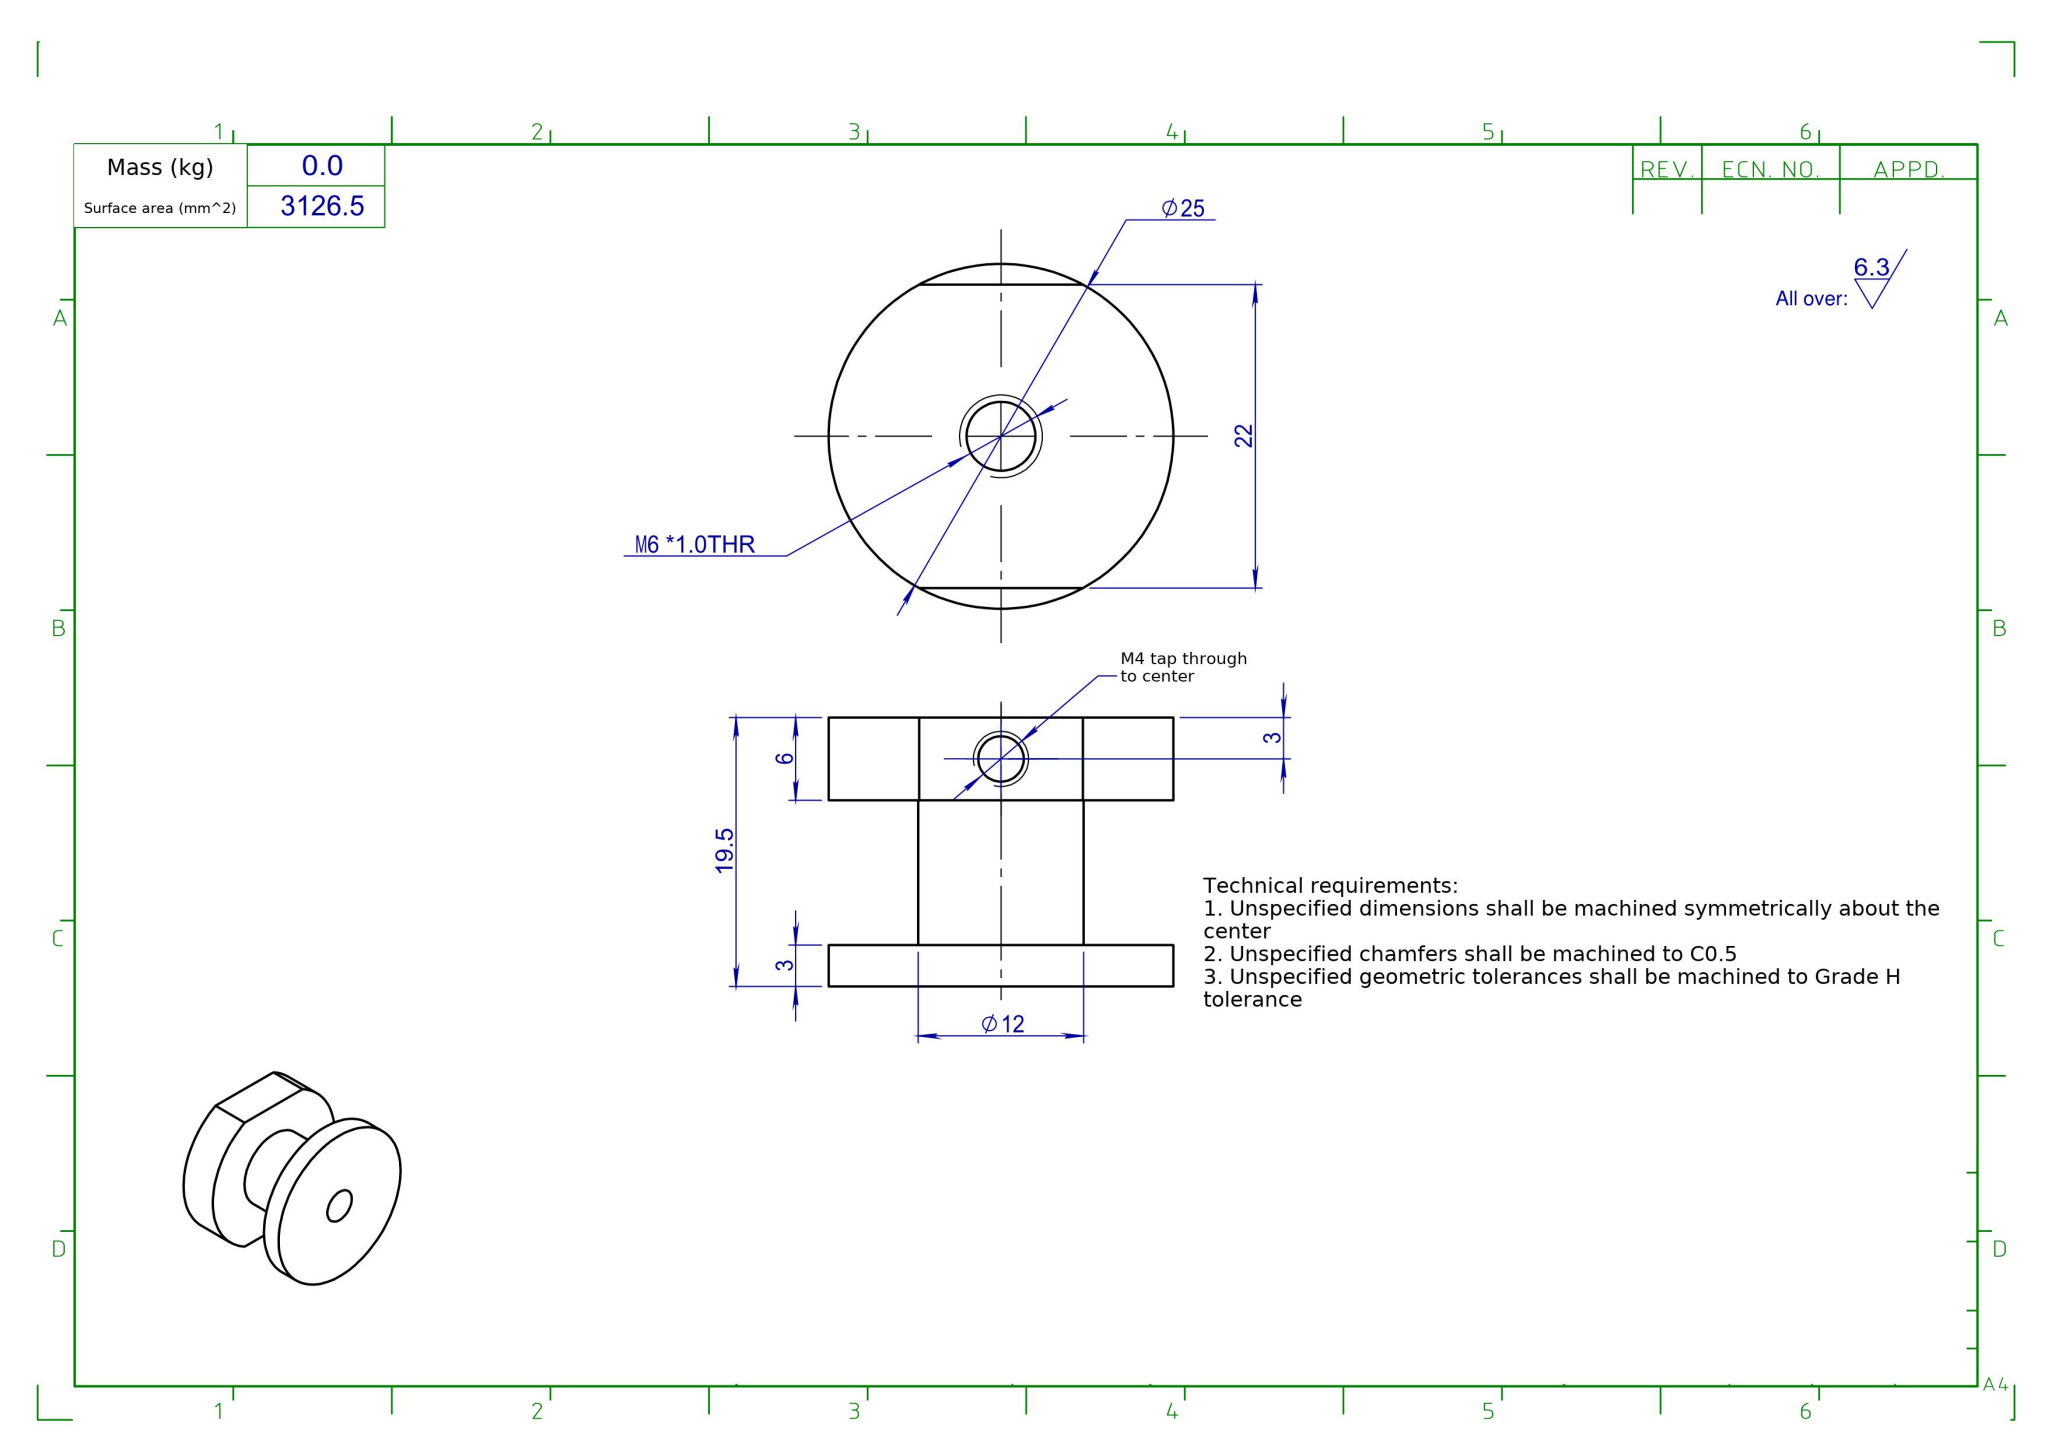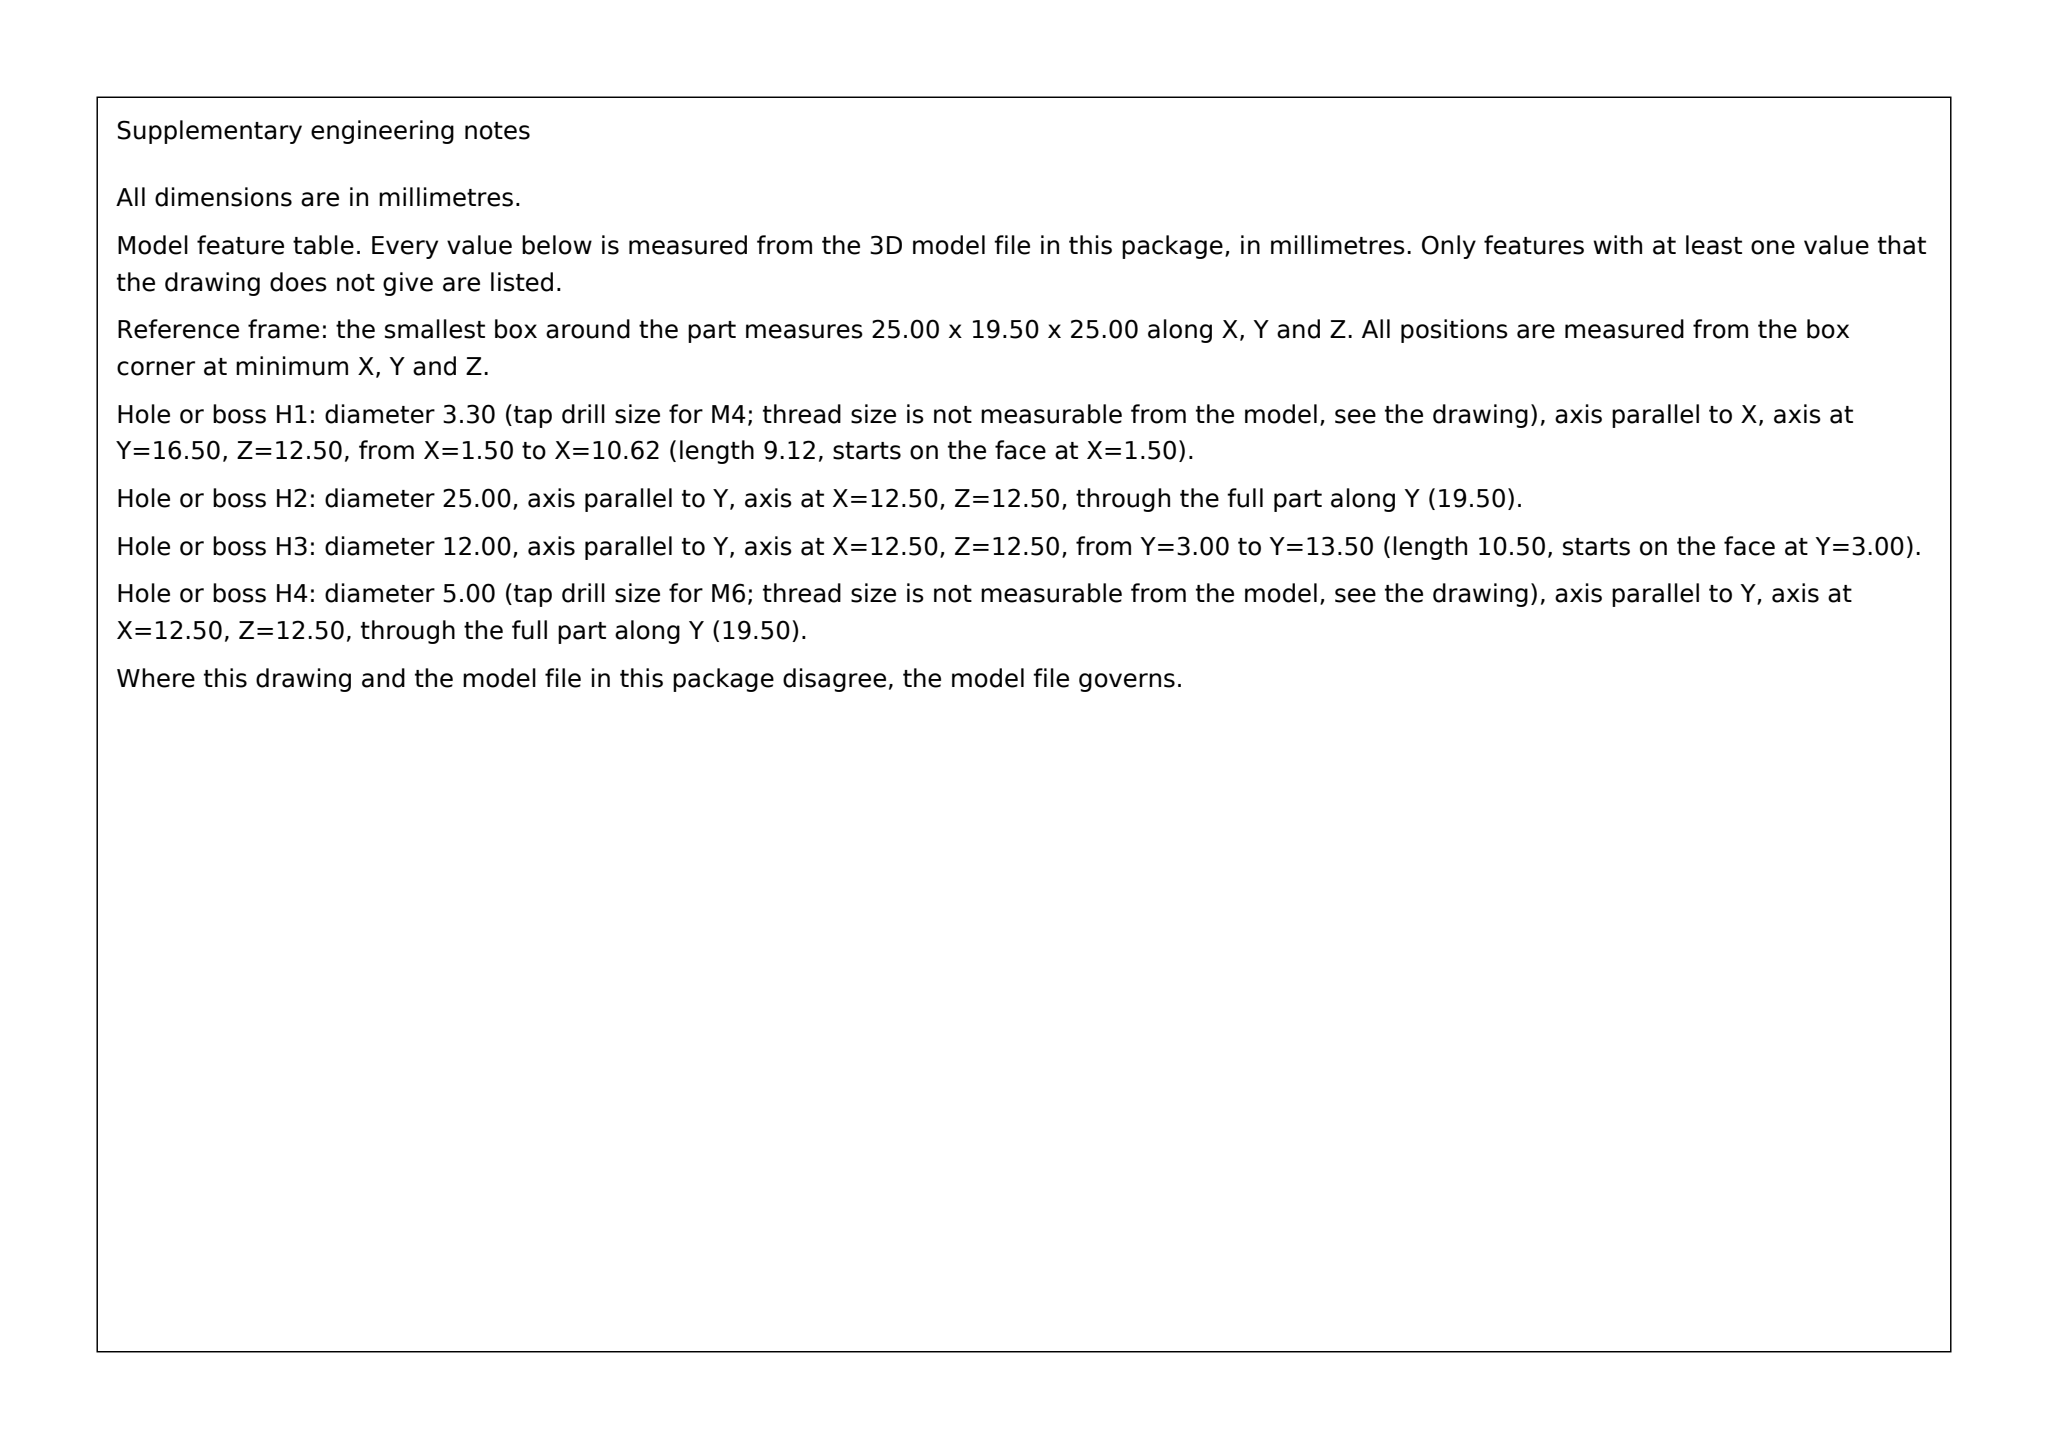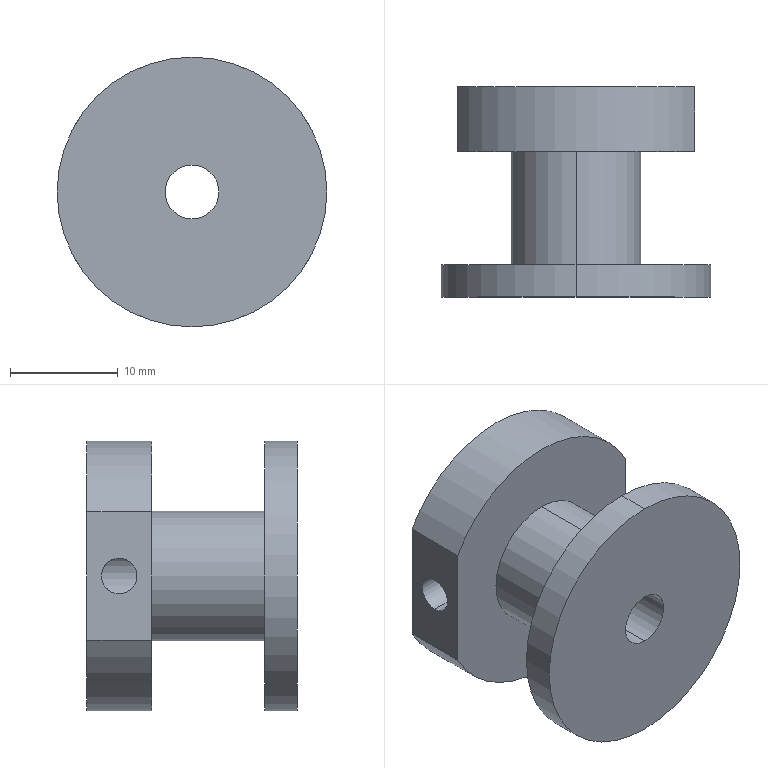Part | SolidWorks | mm | 1 solid | 17 faces | box 25 x 19.5 x 25 mm | volume 5004 mm3 | cylinder 11 | plane 6 | commonest cylinder face diameters 25 x5 3.3 x2 5 x2 12 x2
STEP:
#1=CARTESIAN_POINT('',(-1.878,16.5,-1.65));
#2=VERTEX_POINT('',#1);
#3=CARTESIAN_POINT('',(-1.878,16.5,1.65));
#4=VERTEX_POINT('',#3);
#5=CARTESIAN_POINT('',(-1.878,16.5,-1.65));
#6=CARTESIAN_POINT('',(-1.878,16.277,-1.65));
#7=CARTESIAN_POINT('',(-1.921,16.056,-1.603));
#8=CARTESIAN_POINT('',(-2.049,15.661,-1.437));
#9=CARTESIAN_POINT('',(-2.131,15.485,-1.318));
#10=CARTESIAN_POINT('',(-2.249,15.262,-1.096));
#11=CARTESIAN_POINT('',(-2.286,15.195,-1.016));
#12=CARTESIAN_POINT('',(-2.356,15.077,-0.8415));
#13=CARTESIAN_POINT('',(-2.388,15.025,-0.7465));
#14=CARTESIAN_POINT('',(-2.442,14.939,-0.5467));
#15=CARTESIAN_POINT('',(-2.463,14.907,-0.4426));
#16=CARTESIAN_POINT('',(-2.492,14.862,-0.2252));
#17=CARTESIAN_POINT('',(-2.5,14.85,-0.113));
#18=CARTESIAN_POINT('',(-2.5,14.85,0.109));
#19=CARTESIAN_POINT('',(-2.493,14.861,0.2216));
#20=CARTESIAN_POINT('',(-2.464,14.906,0.439));
#21=CARTESIAN_POINT('',(-2.442,14.938,0.5434));
#22=CARTESIAN_POINT('',(-2.362,15.066,0.8448));
#23=CARTESIAN_POINT('',(-2.288,15.188,1.022));
#24=CARTESIAN_POINT('',(-2.17,15.41,1.243));
#25=CARTESIAN_POINT('',(-2.131,15.491,1.31));
#26=CARTESIAN_POINT('',(-2.054,15.665,1.427));
#27=CARTESIAN_POINT('',(-2.017,15.759,1.478));
#28=CARTESIAN_POINT('',(-1.922,16.053,1.603));
#29=CARTESIAN_POINT('',(-1.878,16.275,1.65));
#30=CARTESIAN_POINT('',(-1.878,16.5,1.65));
#31=B_SPLINE_CURVE_WITH_KNOTS('',3,(#5,#6,#7,#8,#9,#10,#11,#12,#13,#14,#15,#16,#17,#18,#19,#20,#21,#22,#23,#24,#25,#26,#27,#28,#29,#30),.UNSPECIFIED.,.F.,.F.,(4,2,2,2,2,2,2,2,2,2,2,2,4),(0.005325,0.005989,0.006652,0.006984,0.007316,0.007648,0.00798,0.008311,0.008643,0.009307,0.009639,0.00997,0.01063),.UNSPECIFIED.);
#32=EDGE_CURVE('',#2,#4,#31,.T.);
#33=ORIENTED_EDGE('',*,*,#32,.F.);
#34=CARTESIAN_POINT('',(-11.,16.5,-1.65));
#35=VERTEX_POINT('',#34);
#36=CARTESIAN_POINT('',(-11.,16.5,-1.65));
#37=DIRECTION('',(-1.,0.,-0.));
#38=VECTOR('',#37,1000.);
#39=LINE('',#36,#38);
#40=EDGE_CURVE('',#2,#35,#39,.T.);
#41=ORIENTED_EDGE('',*,*,#40,.T.);
#42=CARTESIAN_POINT('',(-11.,16.5,1.65));
#43=VERTEX_POINT('',#42);
#44=CARTESIAN_POINT('',(-11.,16.5,-0.));
#45=DIRECTION('',(-1.,0.,-0.));
#46=DIRECTION('',(0.,0.,1.));
#47=AXIS2_PLACEMENT_3D('',#44,#45,#46);
#48=CIRCLE('',#47,1.65);
#49=EDGE_CURVE('',#35,#43,#48,.T.);
#50=ORIENTED_EDGE('',*,*,#49,.T.);
#51=CARTESIAN_POINT('',(-11.,16.5,1.65));
#52=DIRECTION('',(-1.,0.,-0.));
#53=VECTOR('',#52,1000.);
#54=LINE('',#51,#53);
#55=EDGE_CURVE('',#4,#43,#54,.T.);
#56=ORIENTED_EDGE('',*,*,#55,.F.);
#57=EDGE_LOOP('',(#33,#41,#50,#56));
#58=FACE_OUTER_BOUND('',#57,.T.);
#59=CARTESIAN_POINT('',(-11.,16.5,-0.));
#60=DIRECTION('',(-1.,0.,-0.));
#61=DIRECTION('',(0.,0.,1.));
#62=AXIS2_PLACEMENT_3D('',#59,#60,#61);
#63=CYLINDRICAL_SURFACE('',#62,1.65);
#64=ADVANCED_FACE('',(#58),#63,.F.);
#65=CARTESIAN_POINT('',(-1.878,16.5,1.65));
#66=CARTESIAN_POINT('',(-1.878,16.613,1.65));
#67=CARTESIAN_POINT('',(-1.888,16.723,1.639));
#68=CARTESIAN_POINT('',(-1.926,16.938,1.595));
#69=CARTESIAN_POINT('',(-1.953,17.043,1.562));
#70=CARTESIAN_POINT('',(-2.048,17.339,1.437));
#71=CARTESIAN_POINT('',(-2.131,17.515,1.318));
#72=CARTESIAN_POINT('',(-2.248,17.737,1.097));
#73=CARTESIAN_POINT('',(-2.287,17.805,1.015));
#74=CARTESIAN_POINT('',(-2.356,17.924,0.8403));
#75=CARTESIAN_POINT('',(-2.388,17.975,0.7473));
#76=CARTESIAN_POINT('',(-2.441,18.06,0.5487));
#77=CARTESIAN_POINT('',(-2.463,18.094,0.4419));
#78=CARTESIAN_POINT('',(-2.492,18.138,0.2266));
#79=CARTESIAN_POINT('',(-2.5,18.15,0.1166));
#80=CARTESIAN_POINT('',(-2.5,18.151,-0.2205));
#81=CARTESIAN_POINT('',(-2.469,18.104,-0.4434));
#82=CARTESIAN_POINT('',(-2.363,17.935,-0.8431));
#83=CARTESIAN_POINT('',(-2.288,17.813,-1.021));
#84=CARTESIAN_POINT('',(-2.171,17.59,-1.243));
#85=CARTESIAN_POINT('',(-2.13,17.508,-1.31));
#86=CARTESIAN_POINT('',(-2.054,17.335,-1.427));
#87=CARTESIAN_POINT('',(-2.017,17.243,-1.477));
#88=CARTESIAN_POINT('',(-1.922,16.947,-1.603));
#89=CARTESIAN_POINT('',(-1.878,16.724,-1.65));
#90=CARTESIAN_POINT('',(-1.878,16.5,-1.65));
#91=B_SPLINE_CURVE_WITH_KNOTS('',3,(#65,#66,#67,#68,#69,#70,#71,#72,#73,#74,#75,#76,#77,#78,#79,#80,#81,#82,#83,#84,#85,#86,#87,#88,#89,#90),.UNSPECIFIED.,.F.,.F.,(4,2,2,2,2,2,2,2,2,2,2,2,4),(0.,0.0003328,0.0006656,0.001331,0.001664,0.001997,0.00233,0.002663,0.003328,0.003994,0.004327,0.004659,0.005325),.UNSPECIFIED.);
#92=EDGE_CURVE('',#4,#2,#91,.T.);
#93=ORIENTED_EDGE('',*,*,#92,.T.);
#94=ORIENTED_EDGE('',*,*,#32,.T.);
#95=EDGE_LOOP('',(#93,#94));
#96=FACE_BOUND('',#95,.T.);
#97=CARTESIAN_POINT('',(0.,0.,-2.5));
#98=VERTEX_POINT('',#97);
#99=CARTESIAN_POINT('',(0.,0.,2.5));
#100=VERTEX_POINT('',#99);
#101=CARTESIAN_POINT('',(0.,0.,0.));
#102=DIRECTION('',(0.,1.,0.));
#103=DIRECTION('',(0.,0.,1.));
#104=AXIS2_PLACEMENT_3D('',#101,#102,#103);
#105=CIRCLE('',#104,2.5);
#106=EDGE_CURVE('',#98,#100,#105,.T.);
#107=ORIENTED_EDGE('',*,*,#106,.F.);
#108=CARTESIAN_POINT('',(0.,19.5,-2.5));
#109=VERTEX_POINT('',#108);
#110=CARTESIAN_POINT('',(0.,19.5,-2.5));
#111=DIRECTION('',(0.,1.,0.));
#112=VECTOR('',#111,1000.);
#113=LINE('',#110,#112);
#114=EDGE_CURVE('',#98,#109,#113,.T.);
#115=ORIENTED_EDGE('',*,*,#114,.T.);
#116=CARTESIAN_POINT('',(0.,19.5,2.5));
#117=VERTEX_POINT('',#116);
#118=CARTESIAN_POINT('',(0.,19.5,0.));
#119=DIRECTION('',(0.,1.,0.));
#120=DIRECTION('',(0.,0.,1.));
#121=AXIS2_PLACEMENT_3D('',#118,#119,#120);
#122=CIRCLE('',#121,2.5);
#123=EDGE_CURVE('',#109,#117,#122,.T.);
#124=ORIENTED_EDGE('',*,*,#123,.T.);
#125=CARTESIAN_POINT('',(0.,19.5,2.5));
#126=DIRECTION('',(0.,1.,0.));
#127=VECTOR('',#126,1000.);
#128=LINE('',#125,#127);
#129=EDGE_CURVE('',#100,#117,#128,.T.);
#130=ORIENTED_EDGE('',*,*,#129,.F.);
#131=EDGE_LOOP('',(#107,#115,#124,#130));
#132=FACE_OUTER_BOUND('',#131,.T.);
#133=CARTESIAN_POINT('',(0.,19.5,0.));
#134=DIRECTION('',(0.,1.,0.));
#135=DIRECTION('',(0.,0.,1.));
#136=AXIS2_PLACEMENT_3D('',#133,#134,#135);
#137=CYLINDRICAL_SURFACE('',#136,2.5);
#138=ADVANCED_FACE('',(#96,#132),#137,.F.);
#139=CARTESIAN_POINT('',(0.,13.5,6.));
#140=VERTEX_POINT('',#139);
#141=CARTESIAN_POINT('',(0.,13.5,-6.));
#142=VERTEX_POINT('',#141);
#143=CARTESIAN_POINT('',(0.,13.5,0.));
#144=DIRECTION('',(0.,1.,0.));
#145=DIRECTION('',(0.,0.,1.));
#146=AXIS2_PLACEMENT_3D('',#143,#144,#145);
#147=CIRCLE('',#146,6.);
#148=EDGE_CURVE('',#140,#142,#147,.T.);
#149=ORIENTED_EDGE('',*,*,#148,.F.);
#150=CARTESIAN_POINT('',(0.,3.,6.));
#151=VERTEX_POINT('',#150);
#152=CARTESIAN_POINT('',(0.,13.5,6.));
#153=DIRECTION('',(0.,-1.,0.));
#154=VECTOR('',#153,1000.);
#155=LINE('',#152,#154);
#156=EDGE_CURVE('',#140,#151,#155,.T.);
#157=ORIENTED_EDGE('',*,*,#156,.T.);
#158=CARTESIAN_POINT('',(0.,3.,-6.));
#159=VERTEX_POINT('',#158);
#160=CARTESIAN_POINT('',(0.,3.,0.));
#161=DIRECTION('',(0.,1.,0.));
#162=DIRECTION('',(0.,0.,1.));
#163=AXIS2_PLACEMENT_3D('',#160,#161,#162);
#164=CIRCLE('',#163,6.);
#165=EDGE_CURVE('',#151,#159,#164,.T.);
#166=ORIENTED_EDGE('',*,*,#165,.T.);
#167=CARTESIAN_POINT('',(0.,13.5,-6.));
#168=DIRECTION('',(0.,-1.,0.));
#169=VECTOR('',#168,1000.);
#170=LINE('',#167,#169);
#171=EDGE_CURVE('',#142,#159,#170,.T.);
#172=ORIENTED_EDGE('',*,*,#171,.F.);
#173=EDGE_LOOP('',(#149,#157,#166,#172));
#174=FACE_OUTER_BOUND('',#173,.T.);
#175=CARTESIAN_POINT('',(0.,13.5,0.));
#176=DIRECTION('',(0.,-1.,0.));
#177=DIRECTION('',(0.,0.,-1.));
#178=AXIS2_PLACEMENT_3D('',#175,#176,#177);
#179=CYLINDRICAL_SURFACE('',#178,6.);
#180=ADVANCED_FACE('',(#174),#179,.T.);
#181=CARTESIAN_POINT('',(0.,3.,12.5));
#182=VERTEX_POINT('',#181);
#183=CARTESIAN_POINT('',(0.,3.,-12.5));
#184=VERTEX_POINT('',#183);
#185=CARTESIAN_POINT('',(0.,3.,0.));
#186=DIRECTION('',(0.,1.,0.));
#187=DIRECTION('',(0.,0.,1.));
#188=AXIS2_PLACEMENT_3D('',#185,#186,#187);
#189=CIRCLE('',#188,12.5);
#190=EDGE_CURVE('',#182,#184,#189,.T.);
#191=ORIENTED_EDGE('',*,*,#190,.F.);
#192=CARTESIAN_POINT('',(0.,0.,12.5));
#193=VERTEX_POINT('',#192);
#194=CARTESIAN_POINT('',(0.,3.,12.5));
#195=DIRECTION('',(0.,-1.,0.));
#196=VECTOR('',#195,1000.);
#197=LINE('',#194,#196);
#198=EDGE_CURVE('',#182,#193,#197,.T.);
#199=ORIENTED_EDGE('',*,*,#198,.T.);
#200=CARTESIAN_POINT('',(0.,0.,-12.5));
#201=VERTEX_POINT('',#200);
#202=CARTESIAN_POINT('',(0.,0.,0.));
#203=DIRECTION('',(0.,1.,0.));
#204=DIRECTION('',(0.,0.,1.));
#205=AXIS2_PLACEMENT_3D('',#202,#203,#204);
#206=CIRCLE('',#205,12.5);
#207=EDGE_CURVE('',#193,#201,#206,.T.);
#208=ORIENTED_EDGE('',*,*,#207,.T.);
#209=CARTESIAN_POINT('',(0.,3.,-12.5));
#210=DIRECTION('',(0.,-1.,0.));
#211=VECTOR('',#210,1000.);
#212=LINE('',#209,#211);
#213=EDGE_CURVE('',#184,#201,#212,.T.);
#214=ORIENTED_EDGE('',*,*,#213,.F.);
#215=EDGE_LOOP('',(#191,#199,#208,#214));
#216=FACE_OUTER_BOUND('',#215,.T.);
#217=CARTESIAN_POINT('',(0.,3.,0.));
#218=DIRECTION('',(0.,-1.,0.));
#219=DIRECTION('',(0.,0.,-1.));
#220=AXIS2_PLACEMENT_3D('',#217,#218,#219);
#221=CYLINDRICAL_SURFACE('',#220,12.5);
#222=ADVANCED_FACE('',(#216),#221,.T.);
#223=CARTESIAN_POINT('',(0.,19.5,-12.5));
#224=VERTEX_POINT('',#223);
#225=CARTESIAN_POINT('',(-11.,19.5,-5.937));
#226=VERTEX_POINT('',#225);
#227=CARTESIAN_POINT('',(0.,19.5,0.));
#228=DIRECTION('',(0.,1.,0.));
#229=DIRECTION('',(0.,0.,1.));
#230=AXIS2_PLACEMENT_3D('',#227,#228,#229);
#231=CIRCLE('',#230,12.5);
#232=EDGE_CURVE('',#224,#226,#231,.T.);
#233=ORIENTED_EDGE('',*,*,#232,.F.);
#234=CARTESIAN_POINT('',(0.,13.5,-12.5));
#235=VERTEX_POINT('',#234);
#236=CARTESIAN_POINT('',(0.,19.5,-12.5));
#237=DIRECTION('',(0.,-1.,0.));
#238=VECTOR('',#237,1000.);
#239=LINE('',#236,#238);
#240=EDGE_CURVE('',#224,#235,#239,.T.);
#241=ORIENTED_EDGE('',*,*,#240,.T.);
#242=CARTESIAN_POINT('',(-11.,13.5,-5.937));
#243=VERTEX_POINT('',#242);
#244=CARTESIAN_POINT('',(0.,13.5,0.));
#245=DIRECTION('',(0.,1.,0.));
#246=DIRECTION('',(0.,0.,1.));
#247=AXIS2_PLACEMENT_3D('',#244,#245,#246);
#248=CIRCLE('',#247,12.5);
#249=EDGE_CURVE('',#235,#243,#248,.T.);
#250=ORIENTED_EDGE('',*,*,#249,.T.);
#251=CARTESIAN_POINT('',(-11.,19.5,-5.937));
#252=DIRECTION('',(0.,-1.,0.));
#253=VECTOR('',#252,1000.);
#254=LINE('',#251,#253);
#255=EDGE_CURVE('',#226,#243,#254,.T.);
#256=ORIENTED_EDGE('',*,*,#255,.F.);
#257=EDGE_LOOP('',(#233,#241,#250,#256));
#258=FACE_OUTER_BOUND('',#257,.T.);
#259=CARTESIAN_POINT('',(0.,19.5,0.));
#260=DIRECTION('',(0.,-1.,0.));
#261=DIRECTION('',(0.,0.,-1.));
#262=AXIS2_PLACEMENT_3D('',#259,#260,#261);
#263=CYLINDRICAL_SURFACE('',#262,12.5);
#264=ADVANCED_FACE('',(#258),#263,.T.);
#265=CARTESIAN_POINT('',(0.,13.5,0.));
#266=DIRECTION('',(0.,1.,0.));
#267=DIRECTION('',(0.,0.,1.));
#268=AXIS2_PLACEMENT_3D('',#265,#266,#267);
#269=CIRCLE('',#268,6.);
#270=EDGE_CURVE('',#142,#140,#269,.T.);
#271=ORIENTED_EDGE('',*,*,#270,.T.);
#272=ORIENTED_EDGE('',*,*,#148,.T.);
#273=EDGE_LOOP('',(#271,#272));
#274=FACE_BOUND('',#273,.T.);
#275=CARTESIAN_POINT('',(11.,13.5,5.937));
#276=VERTEX_POINT('',#275);
#277=CARTESIAN_POINT('',(11.,13.5,-5.937));
#278=VERTEX_POINT('',#277);
#279=CARTESIAN_POINT('',(11.,13.5,-0.));
#280=DIRECTION('',(-0.,0.,-1.));
#281=VECTOR('',#280,1000.);
#282=LINE('',#279,#281);
#283=EDGE_CURVE('',#276,#278,#282,.T.);
#284=ORIENTED_EDGE('',*,*,#283,.F.);
#285=CARTESIAN_POINT('',(-11.,13.5,5.937));
#286=VERTEX_POINT('',#285);
#287=CARTESIAN_POINT('',(0.,13.5,0.));
#288=DIRECTION('',(0.,1.,0.));
#289=DIRECTION('',(0.,0.,1.));
#290=AXIS2_PLACEMENT_3D('',#287,#288,#289);
#291=CIRCLE('',#290,12.5);
#292=EDGE_CURVE('',#286,#276,#291,.T.);
#293=ORIENTED_EDGE('',*,*,#292,.F.);
#294=CARTESIAN_POINT('',(-11.,13.5,-0.));
#295=DIRECTION('',(-0.,0.,1.));
#296=VECTOR('',#295,1000.);
#297=LINE('',#294,#296);
#298=EDGE_CURVE('',#243,#286,#297,.T.);
#299=ORIENTED_EDGE('',*,*,#298,.F.);
#300=ORIENTED_EDGE('',*,*,#249,.F.);
#301=CARTESIAN_POINT('',(0.,13.5,0.));
#302=DIRECTION('',(0.,1.,0.));
#303=DIRECTION('',(0.,0.,1.));
#304=AXIS2_PLACEMENT_3D('',#301,#302,#303);
#305=CIRCLE('',#304,12.5);
#306=EDGE_CURVE('',#278,#235,#305,.T.);
#307=ORIENTED_EDGE('',*,*,#306,.F.);
#308=EDGE_LOOP('',(#284,#293,#299,#300,#307));
#309=FACE_OUTER_BOUND('',#308,.T.);
#310=CARTESIAN_POINT('',(0.,13.5,0.));
#311=DIRECTION('',(0.,1.,0.));
#312=DIRECTION('',(0.,0.,1.));
#313=AXIS2_PLACEMENT_3D('',#310,#311,#312);
#314=PLANE('',#313);
#315=ADVANCED_FACE('',(#274,#309),#314,.F.);
#316=CARTESIAN_POINT('',(11.,19.5,5.937));
#317=VERTEX_POINT('',#316);
#318=CARTESIAN_POINT('',(11.,19.5,5.937));
#319=DIRECTION('',(0.,-1.,0.));
#320=VECTOR('',#319,1000.);
#321=LINE('',#318,#320);
#322=EDGE_CURVE('',#317,#276,#321,.T.);
#323=ORIENTED_EDGE('',*,*,#322,.F.);
#324=CARTESIAN_POINT('',(-11.,19.5,5.937));
#325=VERTEX_POINT('',#324);
#326=CARTESIAN_POINT('',(0.,19.5,0.));
#327=DIRECTION('',(0.,1.,0.));
#328=DIRECTION('',(0.,0.,1.));
#329=AXIS2_PLACEMENT_3D('',#326,#327,#328);
#330=CIRCLE('',#329,12.5);
#331=EDGE_CURVE('',#325,#317,#330,.T.);
#332=ORIENTED_EDGE('',*,*,#331,.F.);
#333=CARTESIAN_POINT('',(-11.,19.5,5.937));
#334=DIRECTION('',(0.,1.,0.));
#335=VECTOR('',#334,1000.);
#336=LINE('',#333,#335);
#337=EDGE_CURVE('',#286,#325,#336,.T.);
#338=ORIENTED_EDGE('',*,*,#337,.F.);
#339=ORIENTED_EDGE('',*,*,#292,.T.);
#340=EDGE_LOOP('',(#323,#332,#338,#339));
#341=FACE_OUTER_BOUND('',#340,.T.);
#342=CARTESIAN_POINT('',(0.,19.5,0.));
#343=DIRECTION('',(0.,-1.,0.));
#344=DIRECTION('',(0.,0.,-1.));
#345=AXIS2_PLACEMENT_3D('',#342,#343,#344);
#346=CYLINDRICAL_SURFACE('',#345,12.5);
#347=ADVANCED_FACE('',(#341),#346,.T.);
#348=ORIENTED_EDGE('',*,*,#240,.F.);
#349=CARTESIAN_POINT('',(11.,19.5,-5.937));
#350=VERTEX_POINT('',#349);
#351=CARTESIAN_POINT('',(0.,19.5,0.));
#352=DIRECTION('',(0.,1.,0.));
#353=DIRECTION('',(0.,0.,1.));
#354=AXIS2_PLACEMENT_3D('',#351,#352,#353);
#355=CIRCLE('',#354,12.5);
#356=EDGE_CURVE('',#350,#224,#355,.T.);
#357=ORIENTED_EDGE('',*,*,#356,.F.);
#358=CARTESIAN_POINT('',(11.,19.5,-5.937));
#359=DIRECTION('',(0.,1.,0.));
#360=VECTOR('',#359,1000.);
#361=LINE('',#358,#360);
#362=EDGE_CURVE('',#278,#350,#361,.T.);
#363=ORIENTED_EDGE('',*,*,#362,.F.);
#364=ORIENTED_EDGE('',*,*,#306,.T.);
#365=EDGE_LOOP('',(#348,#357,#363,#364));
#366=FACE_OUTER_BOUND('',#365,.T.);
#367=CARTESIAN_POINT('',(0.,19.5,0.));
#368=DIRECTION('',(0.,-1.,0.));
#369=DIRECTION('',(0.,0.,-1.));
#370=AXIS2_PLACEMENT_3D('',#367,#368,#369);
#371=CYLINDRICAL_SURFACE('',#370,12.5);
#372=ADVANCED_FACE('',(#366),#371,.T.);
#373=CARTESIAN_POINT('',(0.,19.5,0.));
#374=DIRECTION('',(0.,1.,0.));
#375=DIRECTION('',(0.,0.,1.));
#376=AXIS2_PLACEMENT_3D('',#373,#374,#375);
#377=CIRCLE('',#376,2.5);
#378=EDGE_CURVE('',#117,#109,#377,.T.);
#379=ORIENTED_EDGE('',*,*,#378,.F.);
#380=ORIENTED_EDGE('',*,*,#123,.F.);
#381=EDGE_LOOP('',(#379,#380));
#382=FACE_BOUND('',#381,.T.);
#383=ORIENTED_EDGE('',*,*,#331,.T.);
#384=CARTESIAN_POINT('',(11.,19.5,-0.));
#385=DIRECTION('',(-0.,0.,-1.));
#386=VECTOR('',#385,1000.);
#387=LINE('',#384,#386);
#388=EDGE_CURVE('',#317,#350,#387,.T.);
#389=ORIENTED_EDGE('',*,*,#388,.T.);
#390=ORIENTED_EDGE('',*,*,#356,.T.);
#391=ORIENTED_EDGE('',*,*,#232,.T.);
#392=CARTESIAN_POINT('',(-11.,19.5,-0.));
#393=DIRECTION('',(-0.,0.,1.));
#394=VECTOR('',#393,1000.);
#395=LINE('',#392,#394);
#396=EDGE_CURVE('',#226,#325,#395,.T.);
#397=ORIENTED_EDGE('',*,*,#396,.T.);
#398=EDGE_LOOP('',(#383,#389,#390,#391,#397));
#399=FACE_OUTER_BOUND('',#398,.T.);
#400=CARTESIAN_POINT('',(0.,19.5,0.));
#401=DIRECTION('',(0.,1.,0.));
#402=DIRECTION('',(0.,0.,1.));
#403=AXIS2_PLACEMENT_3D('',#400,#401,#402);
#404=PLANE('',#403);
#405=ADVANCED_FACE('',(#382,#399),#404,.T.);
#406=CARTESIAN_POINT('',(0.,3.,0.));
#407=DIRECTION('',(0.,1.,0.));
#408=DIRECTION('',(0.,0.,1.));
#409=AXIS2_PLACEMENT_3D('',#406,#407,#408);
#410=CIRCLE('',#409,12.5);
#411=EDGE_CURVE('',#184,#182,#410,.T.);
#412=ORIENTED_EDGE('',*,*,#411,.T.);
#413=ORIENTED_EDGE('',*,*,#190,.T.);
#414=EDGE_LOOP('',(#412,#413));
#415=FACE_OUTER_BOUND('',#414,.T.);
#416=CARTESIAN_POINT('',(0.,3.,0.));
#417=DIRECTION('',(0.,1.,0.));
#418=DIRECTION('',(0.,0.,1.));
#419=AXIS2_PLACEMENT_3D('',#416,#417,#418);
#420=CIRCLE('',#419,6.);
#421=EDGE_CURVE('',#159,#151,#420,.T.);
#422=ORIENTED_EDGE('',*,*,#421,.F.);
#423=ORIENTED_EDGE('',*,*,#165,.F.);
#424=EDGE_LOOP('',(#422,#423));
#425=FACE_BOUND('',#424,.T.);
#426=CARTESIAN_POINT('',(0.,3.,0.));
#427=DIRECTION('',(0.,1.,0.));
#428=DIRECTION('',(0.,0.,1.));
#429=AXIS2_PLACEMENT_3D('',#426,#427,#428);
#430=PLANE('',#429);
#431=ADVANCED_FACE('',(#415,#425),#430,.T.);
#432=ORIENTED_EDGE('',*,*,#198,.F.);
#433=ORIENTED_EDGE('',*,*,#411,.F.);
#434=ORIENTED_EDGE('',*,*,#213,.T.);
#435=CARTESIAN_POINT('',(0.,0.,0.));
#436=DIRECTION('',(0.,1.,0.));
#437=DIRECTION('',(0.,0.,1.));
#438=AXIS2_PLACEMENT_3D('',#435,#436,#437);
#439=CIRCLE('',#438,12.5);
#440=EDGE_CURVE('',#201,#193,#439,.T.);
#441=ORIENTED_EDGE('',*,*,#440,.T.);
#442=EDGE_LOOP('',(#432,#433,#434,#441));
#443=FACE_OUTER_BOUND('',#442,.T.);
#444=CARTESIAN_POINT('',(0.,3.,0.));
#445=DIRECTION('',(0.,-1.,0.));
#446=DIRECTION('',(0.,0.,-1.));
#447=AXIS2_PLACEMENT_3D('',#444,#445,#446);
#448=CYLINDRICAL_SURFACE('',#447,12.5);
#449=ADVANCED_FACE('',(#443),#448,.T.);
#450=CARTESIAN_POINT('',(0.,0.,0.));
#451=DIRECTION('',(0.,1.,0.));
#452=DIRECTION('',(0.,0.,1.));
#453=AXIS2_PLACEMENT_3D('',#450,#451,#452);
#454=CIRCLE('',#453,2.5);
#455=EDGE_CURVE('',#100,#98,#454,.T.);
#456=ORIENTED_EDGE('',*,*,#455,.T.);
#457=ORIENTED_EDGE('',*,*,#106,.T.);
#458=EDGE_LOOP('',(#456,#457));
#459=FACE_BOUND('',#458,.T.);
#460=ORIENTED_EDGE('',*,*,#440,.F.);
#461=ORIENTED_EDGE('',*,*,#207,.F.);
#462=EDGE_LOOP('',(#460,#461));
#463=FACE_OUTER_BOUND('',#462,.T.);
#464=CARTESIAN_POINT('',(0.,0.,0.));
#465=DIRECTION('',(0.,1.,0.));
#466=DIRECTION('',(0.,0.,1.));
#467=AXIS2_PLACEMENT_3D('',#464,#465,#466);
#468=PLANE('',#467);
#469=ADVANCED_FACE('',(#459,#463),#468,.F.);
#470=ORIENTED_EDGE('',*,*,#156,.F.);
#471=ORIENTED_EDGE('',*,*,#270,.F.);
#472=ORIENTED_EDGE('',*,*,#171,.T.);
#473=ORIENTED_EDGE('',*,*,#421,.T.);
#474=EDGE_LOOP('',(#470,#471,#472,#473));
#475=FACE_OUTER_BOUND('',#474,.T.);
#476=CARTESIAN_POINT('',(0.,13.5,0.));
#477=DIRECTION('',(0.,-1.,0.));
#478=DIRECTION('',(0.,0.,-1.));
#479=AXIS2_PLACEMENT_3D('',#476,#477,#478);
#480=CYLINDRICAL_SURFACE('',#479,6.);
#481=ADVANCED_FACE('',(#475),#480,.T.);
#482=ORIENTED_EDGE('',*,*,#114,.F.);
#483=ORIENTED_EDGE('',*,*,#455,.F.);
#484=ORIENTED_EDGE('',*,*,#129,.T.);
#485=ORIENTED_EDGE('',*,*,#378,.T.);
#486=EDGE_LOOP('',(#482,#483,#484,#485));
#487=FACE_OUTER_BOUND('',#486,.T.);
#488=CARTESIAN_POINT('',(0.,19.5,0.));
#489=DIRECTION('',(0.,1.,0.));
#490=DIRECTION('',(0.,0.,1.));
#491=AXIS2_PLACEMENT_3D('',#488,#489,#490);
#492=CYLINDRICAL_SURFACE('',#491,2.5);
#493=ADVANCED_FACE('',(#487),#492,.F.);
#494=CARTESIAN_POINT('',(-11.,16.5,-0.));
#495=DIRECTION('',(-1.,0.,-0.));
#496=DIRECTION('',(0.,0.,1.));
#497=AXIS2_PLACEMENT_3D('',#494,#495,#496);
#498=CIRCLE('',#497,1.65);
#499=EDGE_CURVE('',#43,#35,#498,.T.);
#500=ORIENTED_EDGE('',*,*,#499,.F.);
#501=ORIENTED_EDGE('',*,*,#49,.F.);
#502=EDGE_LOOP('',(#500,#501));
#503=FACE_BOUND('',#502,.T.);
#504=ORIENTED_EDGE('',*,*,#255,.T.);
#505=ORIENTED_EDGE('',*,*,#298,.T.);
#506=ORIENTED_EDGE('',*,*,#337,.T.);
#507=ORIENTED_EDGE('',*,*,#396,.F.);
#508=EDGE_LOOP('',(#504,#505,#506,#507));
#509=FACE_OUTER_BOUND('',#508,.T.);
#510=CARTESIAN_POINT('',(-11.,-44.642,-18.));
#511=DIRECTION('',(-1.,0.,-0.));
#512=DIRECTION('',(-0.,0.,1.));
#513=AXIS2_PLACEMENT_3D('',#510,#511,#512);
#514=PLANE('',#513);
#515=ADVANCED_FACE('',(#503,#509),#514,.T.);
#516=ORIENTED_EDGE('',*,*,#322,.T.);
#517=ORIENTED_EDGE('',*,*,#283,.T.);
#518=ORIENTED_EDGE('',*,*,#362,.T.);
#519=ORIENTED_EDGE('',*,*,#388,.F.);
#520=EDGE_LOOP('',(#516,#517,#518,#519));
#521=FACE_OUTER_BOUND('',#520,.T.);
#522=CARTESIAN_POINT('',(11.,-44.642,-18.));
#523=DIRECTION('',(1.,0.,-0.));
#524=DIRECTION('',(-0.,0.,-1.));
#525=AXIS2_PLACEMENT_3D('',#522,#523,#524);
#526=PLANE('',#525);
#527=ADVANCED_FACE('',(#521),#526,.T.);
#528=ORIENTED_EDGE('',*,*,#40,.F.);
#529=ORIENTED_EDGE('',*,*,#92,.F.);
#530=ORIENTED_EDGE('',*,*,#55,.T.);
#531=ORIENTED_EDGE('',*,*,#499,.T.);
#532=EDGE_LOOP('',(#528,#529,#530,#531));
#533=FACE_OUTER_BOUND('',#532,.T.);
#534=CARTESIAN_POINT('',(-11.,16.5,-0.));
#535=DIRECTION('',(-1.,0.,-0.));
#536=DIRECTION('',(0.,0.,1.));
#537=AXIS2_PLACEMENT_3D('',#534,#535,#536);
#538=CYLINDRICAL_SURFACE('',#537,1.65);
#539=ADVANCED_FACE('',(#533),#538,.F.);
#540=CLOSED_SHELL('',(#64,#138,#180,#222,#264,#315,#347,#372,#405,#431,#449,#469,#481,#493,#515,#527,#539));
#541=MANIFOLD_SOLID_BREP('',#540);
#542=CARTESIAN_POINT('',(0.,0.,0.));
#543=DIRECTION('',(0.,0.,1.));
#544=DIRECTION('',(1.,0.,0.));
#545=AXIS2_PLACEMENT_3D('',#542,#543,#544);
#546=(LENGTH_UNIT()NAMED_UNIT(*)SI_UNIT(.MILLI.,.METRE.));
#547=UNCERTAINTY_MEASURE_WITH_UNIT(LENGTH_MEASURE(0.00001),#546,'','');
#548=(NAMED_UNIT(*)PLANE_ANGLE_UNIT()SI_UNIT($,.RADIAN.));
#549=(NAMED_UNIT(*)SI_UNIT($,.STERADIAN.)SOLID_ANGLE_UNIT());
#550=(GEOMETRIC_REPRESENTATION_CONTEXT(3)GLOBAL_UNCERTAINTY_ASSIGNED_CONTEXT((#547))GLOBAL_UNIT_ASSIGNED_CONTEXT((#546,#548,#549))REPRESENTATION_CONTEXT('',''));
#551=ADVANCED_BREP_SHAPE_REPRESENTATION('',(#541,#545),#550);